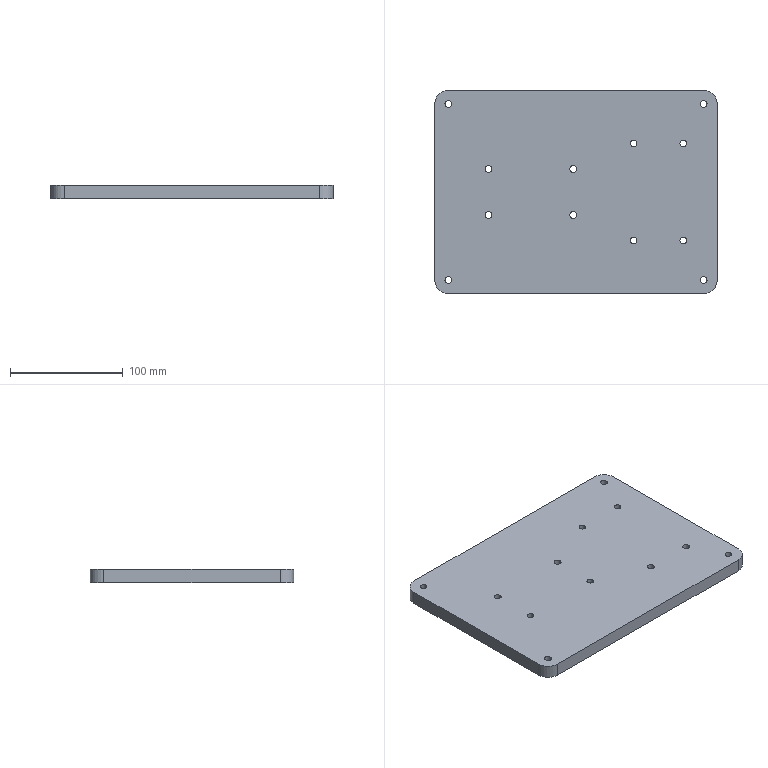Component | NX | BASE_PLATE_2 | 1 solid | 22 faces | volume 534445 mm3 | cylinder 16 | plane 6 | commonest cylinder face diameters 6 x12 24 x4